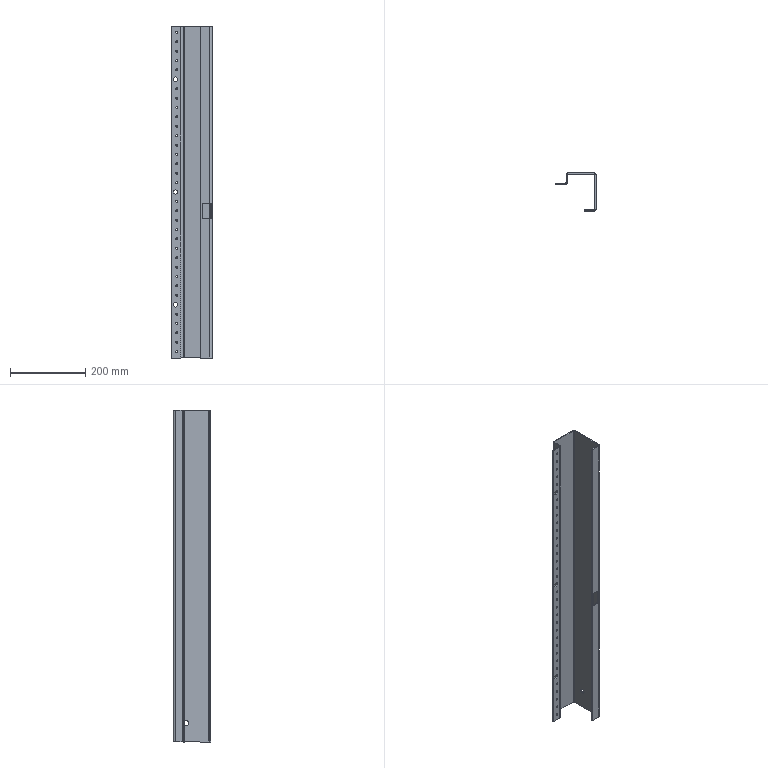Component | SolidWorks | MirrorTopBeamAssembly-2_MirrorUpperBeam-1 | 1 solid | 137 faces | volume 657256 mm3 | cylinder 80 | plane 57 | commonest cylinder face diameters 5.5 x70 6 x4 12 x4 13 x2